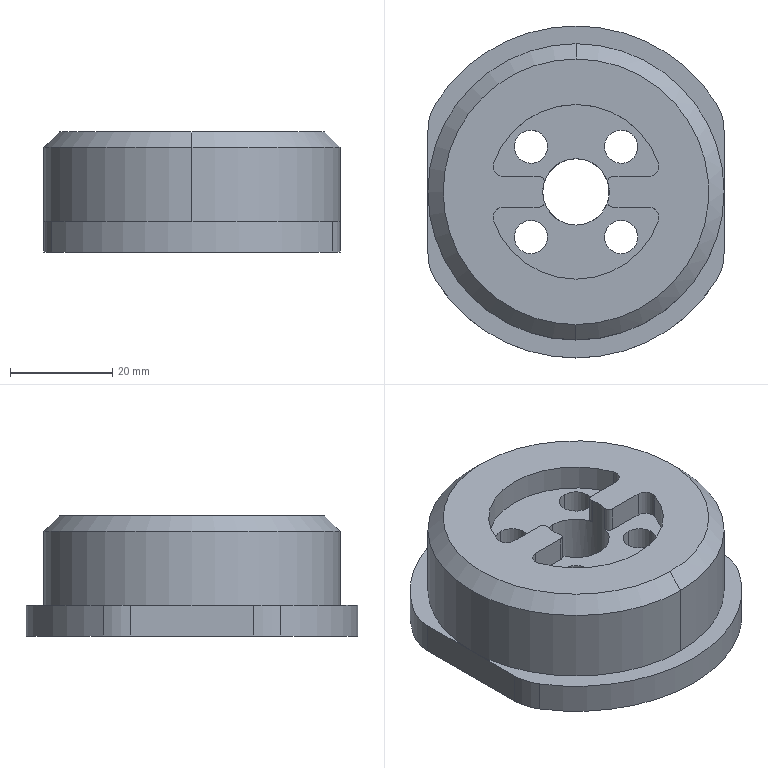CAM job | Mastercam | mm | 10 operations | part box 58 x 65 x 23.5
1. Contour (Ramp) | 9 - 10 平铣刀
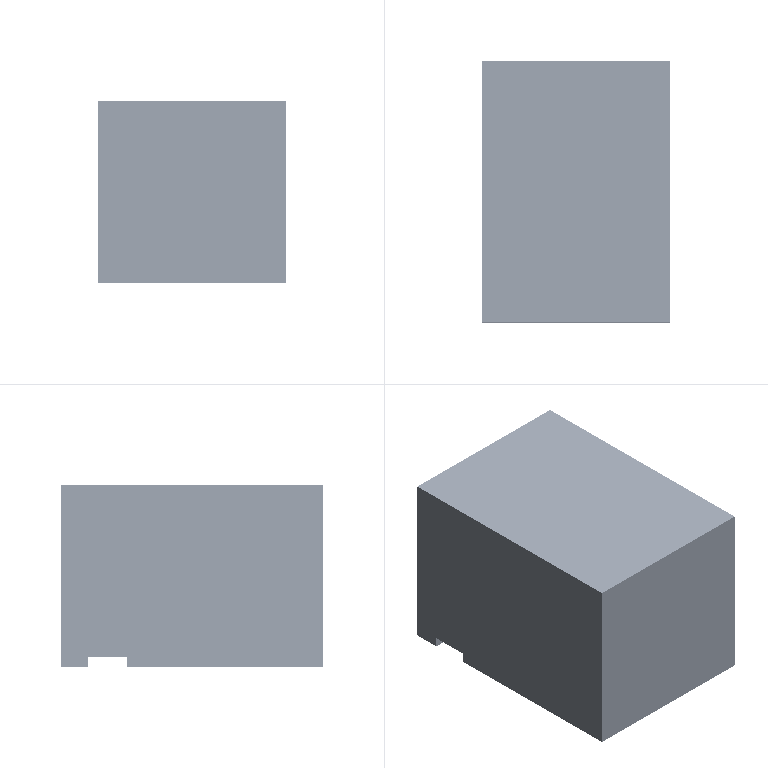2. Contour (2D) | 10 - 10 平铣刀
3. Contour (2D chamfer) | 5 - 4 倒角刀
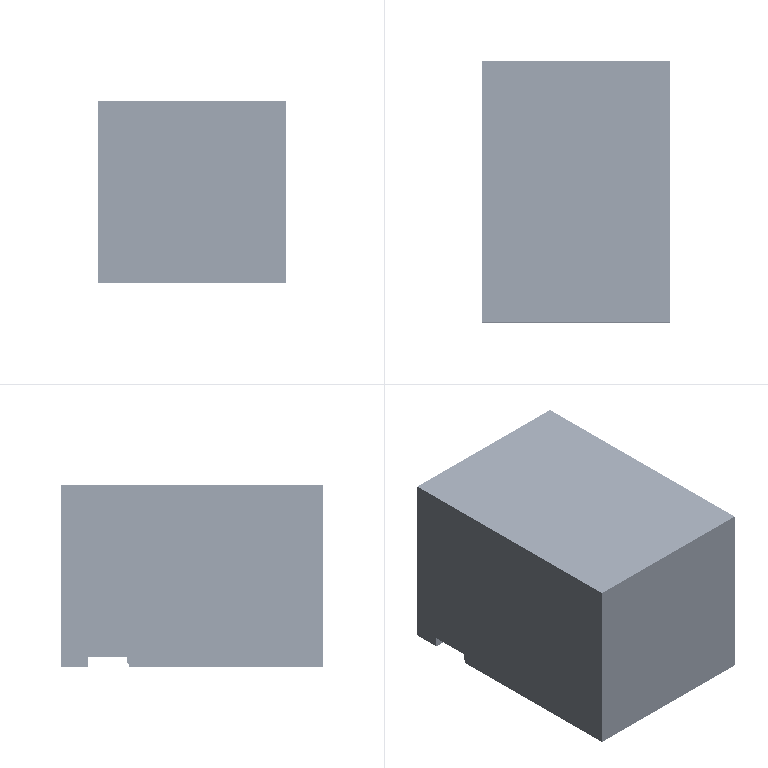4. Drill/Counterbore | 5 - 4 倒角刀
5. 2D High Speed (2D Area Mill) | 8 - 8 平铣刀
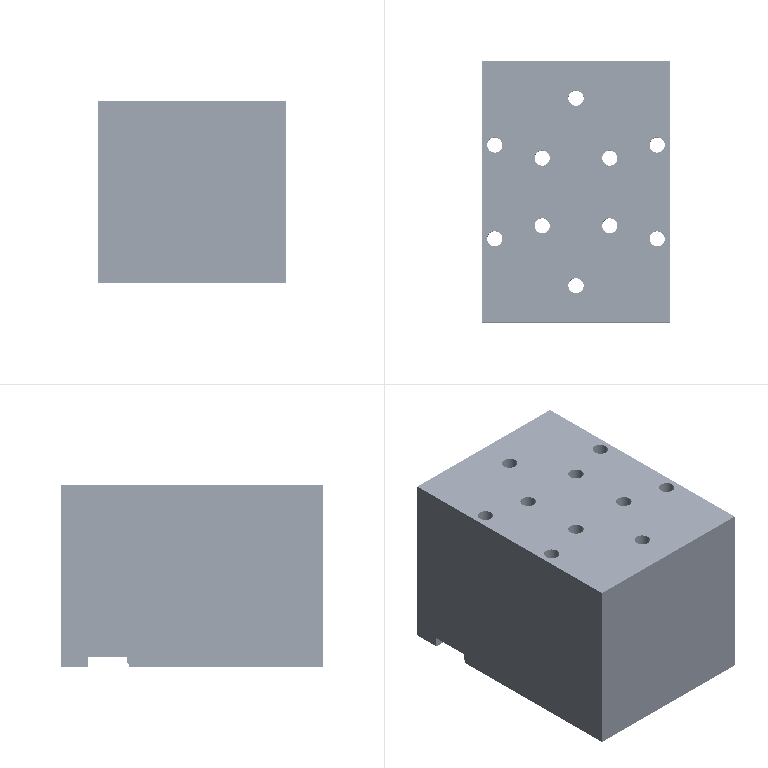6. Contour (Remachining) | 4 - 4 平铣刀
7. 2D High Speed (2D Area Mill) | 4 - 4 平铣刀
8. Contour (2D) | 4 - 4 平铣刀
9. Contour (2D chamfer) | 5 - 4 倒角刀
10. Contour (Ramp) | 14 - 12 平铣刀